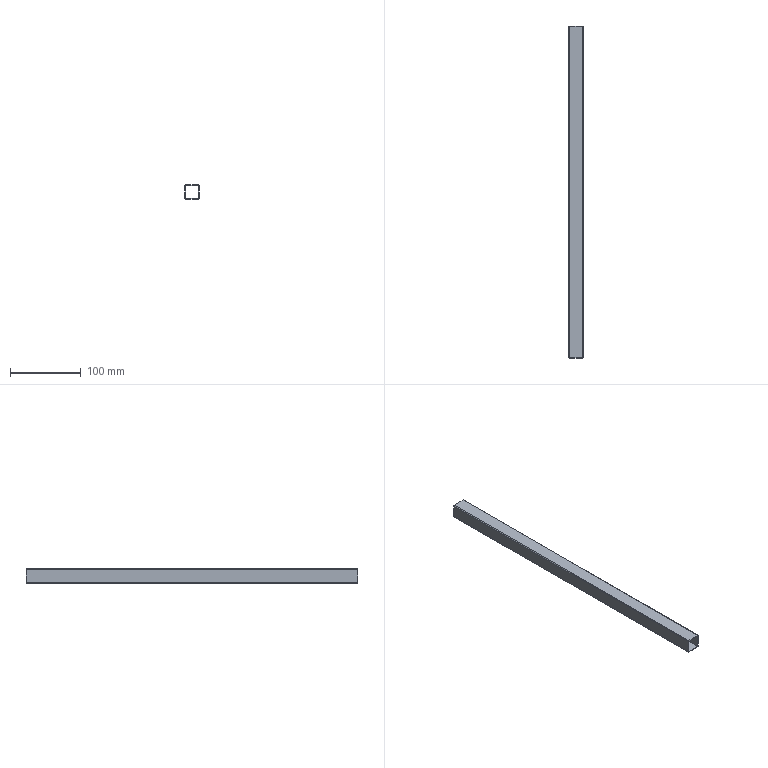Component | SolidWorks | DrawerStiffenerHorizontal-2 | 1 solid | 14 faces | box 20 x 470 x 20 mm | volume 42009 mm3 | plane 10 | cylinder 4 | commonest cylinder face diameters 2 x4
build123d program:
from build123d import *

# Parameters (mm, degrees)
SKETCH1_W           = 17.6
SKETCH1_H           = 17.6
BOSS_EXTRUDE1_DEPTH = 470


with BuildPart() as part:
    # Sketch1 → Boss-Extrude1 (new body)
    with BuildSketch(Plane.XY):
        with BuildLine():
            Line((-9, 10), (9, 10))
            ThreePointArc((9, 10), (9.707, 9.707), (10, 9))
            Line((10, 9), (10, -9))
            ThreePointArc((10, -9), (9.707, -9.707), (9, -10))
            Line((9, -10), (-9, -10))
            ThreePointArc((-9, -10), (-9.707, -9.707), (-10, -9))
            Line((-10, -9), (-10, 9))
            ThreePointArc((-10, 9), (-9.707, 9.707), (-9, 10))
        make_face()
        Rectangle(SKETCH1_W, SKETCH1_H, mode=Mode.SUBTRACT)
    extrude(amount=BOSS_EXTRUDE1_DEPTH)


solid = part.part

# Placed as in the assembly
solid = solid.moved(Location((8.5, 236, 110), (90, 0, 0)))
STEP:
#1=CARTESIAN_POINT('',(0.7283,-9.213,4.685));
#2=VERTEX_POINT('',#1);
#3=CARTESIAN_POINT('',(0.689,-9.213,4.724));
#4=VERTEX_POINT('',#3);
#5=CARTESIAN_POINT('',(0.689,-9.213,4.685));
#6=DIRECTION('',(-0.,-1.,-0.));
#7=DIRECTION('',(0.,0.,-1.));
#8=AXIS2_PLACEMENT_3D('',#5,#6,#7);
#9=CIRCLE('',#8,0.03937);
#10=EDGE_CURVE('',#2,#4,#9,.T.);
#11=ORIENTED_EDGE('',*,*,#10,.T.);
#12=CARTESIAN_POINT('',(-0.01969,-9.213,4.724));
#13=VERTEX_POINT('',#12);
#14=CARTESIAN_POINT('',(0.689,-9.213,4.724));
#15=DIRECTION('',(-1.,-0.,-0.));
#16=VECTOR('',#15,39.37);
#17=LINE('',#14,#16);
#18=EDGE_CURVE('',#4,#13,#17,.T.);
#19=ORIENTED_EDGE('',*,*,#18,.T.);
#20=CARTESIAN_POINT('',(-0.05906,-9.213,4.685));
#21=VERTEX_POINT('',#20);
#22=CARTESIAN_POINT('',(-0.01969,-9.213,4.685));
#23=DIRECTION('',(-0.,-1.,-0.));
#24=DIRECTION('',(0.,0.,1.));
#25=AXIS2_PLACEMENT_3D('',#22,#23,#24);
#26=CIRCLE('',#25,0.03937);
#27=EDGE_CURVE('',#13,#21,#26,.T.);
#28=ORIENTED_EDGE('',*,*,#27,.T.);
#29=CARTESIAN_POINT('',(-0.05906,-9.213,3.976));
#30=VERTEX_POINT('',#29);
#31=CARTESIAN_POINT('',(-0.05906,-9.213,4.685));
#32=DIRECTION('',(-0.,0.,-1.));
#33=VECTOR('',#32,39.37);
#34=LINE('',#31,#33);
#35=EDGE_CURVE('',#21,#30,#34,.T.);
#36=ORIENTED_EDGE('',*,*,#35,.T.);
#37=CARTESIAN_POINT('',(-0.01969,-9.213,3.937));
#38=VERTEX_POINT('',#37);
#39=CARTESIAN_POINT('',(-0.01969,-9.213,3.976));
#40=DIRECTION('',(-0.,-1.,-0.));
#41=DIRECTION('',(0.,0.,-1.));
#42=AXIS2_PLACEMENT_3D('',#39,#40,#41);
#43=CIRCLE('',#42,0.03937);
#44=EDGE_CURVE('',#30,#38,#43,.T.);
#45=ORIENTED_EDGE('',*,*,#44,.T.);
#46=CARTESIAN_POINT('',(0.689,-9.213,3.937));
#47=VERTEX_POINT('',#46);
#48=CARTESIAN_POINT('',(0.689,-9.213,3.937));
#49=DIRECTION('',(1.,0.,0.));
#50=VECTOR('',#49,39.37);
#51=LINE('',#48,#50);
#52=EDGE_CURVE('',#38,#47,#51,.T.);
#53=ORIENTED_EDGE('',*,*,#52,.T.);
#54=CARTESIAN_POINT('',(0.7283,-9.213,3.976));
#55=VERTEX_POINT('',#54);
#56=CARTESIAN_POINT('',(0.689,-9.213,3.976));
#57=DIRECTION('',(-0.,-1.,-0.));
#58=DIRECTION('',(0.,0.,-1.));
#59=AXIS2_PLACEMENT_3D('',#56,#57,#58);
#60=CIRCLE('',#59,0.03937);
#61=EDGE_CURVE('',#47,#55,#60,.T.);
#62=ORIENTED_EDGE('',*,*,#61,.T.);
#63=CARTESIAN_POINT('',(0.7283,-9.213,4.685));
#64=DIRECTION('',(0.,-0.,1.));
#65=VECTOR('',#64,39.37);
#66=LINE('',#63,#65);
#67=EDGE_CURVE('',#55,#2,#66,.T.);
#68=ORIENTED_EDGE('',*,*,#67,.T.);
#69=EDGE_LOOP('',(#11,#19,#28,#36,#45,#53,#62,#68));
#70=FACE_OUTER_BOUND('',#69,.T.);
#71=CARTESIAN_POINT('',(0.6811,-9.213,4.677));
#72=VERTEX_POINT('',#71);
#73=CARTESIAN_POINT('',(-0.01181,-9.213,4.677));
#74=VERTEX_POINT('',#73);
#75=CARTESIAN_POINT('',(0.6811,-9.213,4.677));
#76=DIRECTION('',(-1.,-0.,-0.));
#77=VECTOR('',#76,39.37);
#78=LINE('',#75,#77);
#79=EDGE_CURVE('',#72,#74,#78,.T.);
#80=ORIENTED_EDGE('',*,*,#79,.F.);
#81=CARTESIAN_POINT('',(0.6811,-9.213,3.984));
#82=VERTEX_POINT('',#81);
#83=CARTESIAN_POINT('',(0.6811,-9.213,4.677));
#84=DIRECTION('',(0.,-0.,1.));
#85=VECTOR('',#84,39.37);
#86=LINE('',#83,#85);
#87=EDGE_CURVE('',#82,#72,#86,.T.);
#88=ORIENTED_EDGE('',*,*,#87,.F.);
#89=CARTESIAN_POINT('',(-0.01181,-9.213,3.984));
#90=VERTEX_POINT('',#89);
#91=CARTESIAN_POINT('',(0.6811,-9.213,3.984));
#92=DIRECTION('',(1.,0.,0.));
#93=VECTOR('',#92,39.37);
#94=LINE('',#91,#93);
#95=EDGE_CURVE('',#90,#82,#94,.T.);
#96=ORIENTED_EDGE('',*,*,#95,.F.);
#97=CARTESIAN_POINT('',(-0.01181,-9.213,4.677));
#98=DIRECTION('',(-0.,0.,-1.));
#99=VECTOR('',#98,39.37);
#100=LINE('',#97,#99);
#101=EDGE_CURVE('',#74,#90,#100,.T.);
#102=ORIENTED_EDGE('',*,*,#101,.F.);
#103=EDGE_LOOP('',(#80,#88,#96,#102));
#104=FACE_BOUND('',#103,.T.);
#105=CARTESIAN_POINT('',(0.689,-9.213,4.685));
#106=DIRECTION('',(-0.,-1.,-0.));
#107=DIRECTION('',(-0.,0.,-1.));
#108=AXIS2_PLACEMENT_3D('',#105,#106,#107);
#109=PLANE('',#108);
#110=ADVANCED_FACE('',(#70,#104),#109,.T.);
#111=CARTESIAN_POINT('',(0.7283,9.291,4.685));
#112=VERTEX_POINT('',#111);
#113=CARTESIAN_POINT('',(0.689,9.291,4.724));
#114=VERTEX_POINT('',#113);
#115=CARTESIAN_POINT('',(0.689,9.291,4.685));
#116=DIRECTION('',(-0.,-1.,-0.));
#117=DIRECTION('',(0.,0.,-1.));
#118=AXIS2_PLACEMENT_3D('',#115,#116,#117);
#119=CIRCLE('',#118,0.03937);
#120=EDGE_CURVE('',#112,#114,#119,.T.);
#121=ORIENTED_EDGE('',*,*,#120,.F.);
#122=CARTESIAN_POINT('',(0.7283,9.291,3.976));
#123=VERTEX_POINT('',#122);
#124=CARTESIAN_POINT('',(0.7283,9.291,4.685));
#125=DIRECTION('',(0.,-0.,1.));
#126=VECTOR('',#125,39.37);
#127=LINE('',#124,#126);
#128=EDGE_CURVE('',#123,#112,#127,.T.);
#129=ORIENTED_EDGE('',*,*,#128,.F.);
#130=CARTESIAN_POINT('',(0.689,9.291,3.937));
#131=VERTEX_POINT('',#130);
#132=CARTESIAN_POINT('',(0.689,9.291,3.976));
#133=DIRECTION('',(-0.,-1.,-0.));
#134=DIRECTION('',(0.,0.,-1.));
#135=AXIS2_PLACEMENT_3D('',#132,#133,#134);
#136=CIRCLE('',#135,0.03937);
#137=EDGE_CURVE('',#131,#123,#136,.T.);
#138=ORIENTED_EDGE('',*,*,#137,.F.);
#139=CARTESIAN_POINT('',(-0.01969,9.291,3.937));
#140=VERTEX_POINT('',#139);
#141=CARTESIAN_POINT('',(0.689,9.291,3.937));
#142=DIRECTION('',(1.,0.,0.));
#143=VECTOR('',#142,39.37);
#144=LINE('',#141,#143);
#145=EDGE_CURVE('',#140,#131,#144,.T.);
#146=ORIENTED_EDGE('',*,*,#145,.F.);
#147=CARTESIAN_POINT('',(-0.05906,9.291,3.976));
#148=VERTEX_POINT('',#147);
#149=CARTESIAN_POINT('',(-0.01969,9.291,3.976));
#150=DIRECTION('',(-0.,-1.,-0.));
#151=DIRECTION('',(0.,0.,-1.));
#152=AXIS2_PLACEMENT_3D('',#149,#150,#151);
#153=CIRCLE('',#152,0.03937);
#154=EDGE_CURVE('',#148,#140,#153,.T.);
#155=ORIENTED_EDGE('',*,*,#154,.F.);
#156=CARTESIAN_POINT('',(-0.05906,9.291,4.685));
#157=VERTEX_POINT('',#156);
#158=CARTESIAN_POINT('',(-0.05906,9.291,4.685));
#159=DIRECTION('',(-0.,0.,-1.));
#160=VECTOR('',#159,39.37);
#161=LINE('',#158,#160);
#162=EDGE_CURVE('',#157,#148,#161,.T.);
#163=ORIENTED_EDGE('',*,*,#162,.F.);
#164=CARTESIAN_POINT('',(-0.01969,9.291,4.724));
#165=VERTEX_POINT('',#164);
#166=CARTESIAN_POINT('',(-0.01969,9.291,4.685));
#167=DIRECTION('',(-0.,-1.,-0.));
#168=DIRECTION('',(0.,0.,1.));
#169=AXIS2_PLACEMENT_3D('',#166,#167,#168);
#170=CIRCLE('',#169,0.03937);
#171=EDGE_CURVE('',#165,#157,#170,.T.);
#172=ORIENTED_EDGE('',*,*,#171,.F.);
#173=CARTESIAN_POINT('',(0.689,9.291,4.724));
#174=DIRECTION('',(-1.,-0.,-0.));
#175=VECTOR('',#174,39.37);
#176=LINE('',#173,#175);
#177=EDGE_CURVE('',#114,#165,#176,.T.);
#178=ORIENTED_EDGE('',*,*,#177,.F.);
#179=EDGE_LOOP('',(#121,#129,#138,#146,#155,#163,#172,#178));
#180=FACE_OUTER_BOUND('',#179,.T.);
#181=CARTESIAN_POINT('',(0.6811,9.291,3.984));
#182=VERTEX_POINT('',#181);
#183=CARTESIAN_POINT('',(0.6811,9.291,4.677));
#184=VERTEX_POINT('',#183);
#185=CARTESIAN_POINT('',(0.6811,9.291,4.677));
#186=DIRECTION('',(0.,-0.,1.));
#187=VECTOR('',#186,39.37);
#188=LINE('',#185,#187);
#189=EDGE_CURVE('',#182,#184,#188,.T.);
#190=ORIENTED_EDGE('',*,*,#189,.T.);
#191=CARTESIAN_POINT('',(-0.01181,9.291,4.677));
#192=VERTEX_POINT('',#191);
#193=CARTESIAN_POINT('',(0.6811,9.291,4.677));
#194=DIRECTION('',(-1.,-0.,-0.));
#195=VECTOR('',#194,39.37);
#196=LINE('',#193,#195);
#197=EDGE_CURVE('',#184,#192,#196,.T.);
#198=ORIENTED_EDGE('',*,*,#197,.T.);
#199=CARTESIAN_POINT('',(-0.01181,9.291,3.984));
#200=VERTEX_POINT('',#199);
#201=CARTESIAN_POINT('',(-0.01181,9.291,4.677));
#202=DIRECTION('',(-0.,0.,-1.));
#203=VECTOR('',#202,39.37);
#204=LINE('',#201,#203);
#205=EDGE_CURVE('',#192,#200,#204,.T.);
#206=ORIENTED_EDGE('',*,*,#205,.T.);
#207=CARTESIAN_POINT('',(0.6811,9.291,3.984));
#208=DIRECTION('',(1.,0.,0.));
#209=VECTOR('',#208,39.37);
#210=LINE('',#207,#209);
#211=EDGE_CURVE('',#200,#182,#210,.T.);
#212=ORIENTED_EDGE('',*,*,#211,.T.);
#213=EDGE_LOOP('',(#190,#198,#206,#212));
#214=FACE_BOUND('',#213,.T.);
#215=CARTESIAN_POINT('',(0.689,9.291,4.685));
#216=DIRECTION('',(-0.,-1.,-0.));
#217=DIRECTION('',(-0.,0.,-1.));
#218=AXIS2_PLACEMENT_3D('',#215,#216,#217);
#219=PLANE('',#218);
#220=ADVANCED_FACE('',(#180,#214),#219,.F.);
#221=ORIENTED_EDGE('',*,*,#120,.T.);
#222=CARTESIAN_POINT('',(0.689,-9.213,4.724));
#223=DIRECTION('',(0.,1.,0.));
#224=VECTOR('',#223,39.37);
#225=LINE('',#222,#224);
#226=EDGE_CURVE('',#4,#114,#225,.T.);
#227=ORIENTED_EDGE('',*,*,#226,.F.);
#228=ORIENTED_EDGE('',*,*,#10,.F.);
#229=CARTESIAN_POINT('',(0.7283,-9.213,4.685));
#230=DIRECTION('',(0.,1.,0.));
#231=VECTOR('',#230,39.37);
#232=LINE('',#229,#231);
#233=EDGE_CURVE('',#2,#112,#232,.T.);
#234=ORIENTED_EDGE('',*,*,#233,.T.);
#235=EDGE_LOOP('',(#221,#227,#228,#234));
#236=FACE_OUTER_BOUND('',#235,.T.);
#237=CARTESIAN_POINT('',(0.689,-9.213,4.685));
#238=DIRECTION('',(0.,1.,0.));
#239=DIRECTION('',(0.,0.,1.));
#240=AXIS2_PLACEMENT_3D('',#237,#238,#239);
#241=CYLINDRICAL_SURFACE('',#240,0.03937);
#242=ADVANCED_FACE('',(#236),#241,.T.);
#243=ORIENTED_EDGE('',*,*,#177,.T.);
#244=CARTESIAN_POINT('',(-0.01969,-9.213,4.724));
#245=DIRECTION('',(0.,1.,0.));
#246=VECTOR('',#245,39.37);
#247=LINE('',#244,#246);
#248=EDGE_CURVE('',#13,#165,#247,.T.);
#249=ORIENTED_EDGE('',*,*,#248,.F.);
#250=ORIENTED_EDGE('',*,*,#18,.F.);
#251=ORIENTED_EDGE('',*,*,#226,.T.);
#252=EDGE_LOOP('',(#243,#249,#250,#251));
#253=FACE_OUTER_BOUND('',#252,.T.);
#254=CARTESIAN_POINT('',(0.689,-9.213,4.724));
#255=DIRECTION('',(-0.,0.,-1.));
#256=DIRECTION('',(0.,1.,0.));
#257=AXIS2_PLACEMENT_3D('',#254,#255,#256);
#258=PLANE('',#257);
#259=ADVANCED_FACE('',(#253),#258,.F.);
#260=ORIENTED_EDGE('',*,*,#171,.T.);
#261=CARTESIAN_POINT('',(-0.05906,-9.213,4.685));
#262=DIRECTION('',(0.,1.,0.));
#263=VECTOR('',#262,39.37);
#264=LINE('',#261,#263);
#265=EDGE_CURVE('',#21,#157,#264,.T.);
#266=ORIENTED_EDGE('',*,*,#265,.F.);
#267=ORIENTED_EDGE('',*,*,#27,.F.);
#268=ORIENTED_EDGE('',*,*,#248,.T.);
#269=EDGE_LOOP('',(#260,#266,#267,#268));
#270=FACE_OUTER_BOUND('',#269,.T.);
#271=CARTESIAN_POINT('',(-0.01969,-9.213,4.685));
#272=DIRECTION('',(0.,1.,0.));
#273=DIRECTION('',(0.,0.,1.));
#274=AXIS2_PLACEMENT_3D('',#271,#272,#273);
#275=CYLINDRICAL_SURFACE('',#274,0.03937);
#276=ADVANCED_FACE('',(#270),#275,.T.);
#277=ORIENTED_EDGE('',*,*,#162,.T.);
#278=CARTESIAN_POINT('',(-0.05906,-9.213,3.976));
#279=DIRECTION('',(0.,1.,0.));
#280=VECTOR('',#279,39.37);
#281=LINE('',#278,#280);
#282=EDGE_CURVE('',#30,#148,#281,.T.);
#283=ORIENTED_EDGE('',*,*,#282,.F.);
#284=ORIENTED_EDGE('',*,*,#35,.F.);
#285=ORIENTED_EDGE('',*,*,#265,.T.);
#286=EDGE_LOOP('',(#277,#283,#284,#285));
#287=FACE_OUTER_BOUND('',#286,.T.);
#288=CARTESIAN_POINT('',(-0.05906,-9.213,4.685));
#289=DIRECTION('',(1.,-0.,0.));
#290=DIRECTION('',(-0.,-1.,-0.));
#291=AXIS2_PLACEMENT_3D('',#288,#289,#290);
#292=PLANE('',#291);
#293=ADVANCED_FACE('',(#287),#292,.F.);
#294=ORIENTED_EDGE('',*,*,#154,.T.);
#295=CARTESIAN_POINT('',(-0.01969,-9.213,3.937));
#296=DIRECTION('',(0.,1.,0.));
#297=VECTOR('',#296,39.37);
#298=LINE('',#295,#297);
#299=EDGE_CURVE('',#38,#140,#298,.T.);
#300=ORIENTED_EDGE('',*,*,#299,.F.);
#301=ORIENTED_EDGE('',*,*,#44,.F.);
#302=ORIENTED_EDGE('',*,*,#282,.T.);
#303=EDGE_LOOP('',(#294,#300,#301,#302));
#304=FACE_OUTER_BOUND('',#303,.T.);
#305=CARTESIAN_POINT('',(-0.01969,-9.213,3.976));
#306=DIRECTION('',(0.,1.,0.));
#307=DIRECTION('',(0.,0.,1.));
#308=AXIS2_PLACEMENT_3D('',#305,#306,#307);
#309=CYLINDRICAL_SURFACE('',#308,0.03937);
#310=ADVANCED_FACE('',(#304),#309,.T.);
#311=ORIENTED_EDGE('',*,*,#145,.T.);
#312=CARTESIAN_POINT('',(0.689,-9.213,3.937));
#313=DIRECTION('',(0.,1.,0.));
#314=VECTOR('',#313,39.37);
#315=LINE('',#312,#314);
#316=EDGE_CURVE('',#47,#131,#315,.T.);
#317=ORIENTED_EDGE('',*,*,#316,.F.);
#318=ORIENTED_EDGE('',*,*,#52,.F.);
#319=ORIENTED_EDGE('',*,*,#299,.T.);
#320=EDGE_LOOP('',(#311,#317,#318,#319));
#321=FACE_OUTER_BOUND('',#320,.T.);
#322=CARTESIAN_POINT('',(0.689,-9.213,3.937));
#323=DIRECTION('',(-0.,-0.,1.));
#324=DIRECTION('',(-1.,-0.,-0.));
#325=AXIS2_PLACEMENT_3D('',#322,#323,#324);
#326=PLANE('',#325);
#327=ADVANCED_FACE('',(#321),#326,.F.);
#328=ORIENTED_EDGE('',*,*,#137,.T.);
#329=CARTESIAN_POINT('',(0.7283,-9.213,3.976));
#330=DIRECTION('',(0.,1.,0.));
#331=VECTOR('',#330,39.37);
#332=LINE('',#329,#331);
#333=EDGE_CURVE('',#55,#123,#332,.T.);
#334=ORIENTED_EDGE('',*,*,#333,.F.);
#335=ORIENTED_EDGE('',*,*,#61,.F.);
#336=ORIENTED_EDGE('',*,*,#316,.T.);
#337=EDGE_LOOP('',(#328,#334,#335,#336));
#338=FACE_OUTER_BOUND('',#337,.T.);
#339=CARTESIAN_POINT('',(0.689,-9.213,3.976));
#340=DIRECTION('',(0.,1.,0.));
#341=DIRECTION('',(0.,0.,1.));
#342=AXIS2_PLACEMENT_3D('',#339,#340,#341);
#343=CYLINDRICAL_SURFACE('',#342,0.03937);
#344=ADVANCED_FACE('',(#338),#343,.T.);
#345=ORIENTED_EDGE('',*,*,#128,.T.);
#346=ORIENTED_EDGE('',*,*,#233,.F.);
#347=ORIENTED_EDGE('',*,*,#67,.F.);
#348=ORIENTED_EDGE('',*,*,#333,.T.);
#349=EDGE_LOOP('',(#345,#346,#347,#348));
#350=FACE_OUTER_BOUND('',#349,.T.);
#351=CARTESIAN_POINT('',(0.7283,-9.213,4.685));
#352=DIRECTION('',(-1.,0.,-0.));
#353=DIRECTION('',(0.,1.,0.));
#354=AXIS2_PLACEMENT_3D('',#351,#352,#353);
#355=PLANE('',#354);
#356=ADVANCED_FACE('',(#350),#355,.F.);
#357=ORIENTED_EDGE('',*,*,#189,.F.);
#358=CARTESIAN_POINT('',(0.6811,-9.213,3.984));
#359=DIRECTION('',(0.,1.,0.));
#360=VECTOR('',#359,39.37);
#361=LINE('',#358,#360);
#362=EDGE_CURVE('',#82,#182,#361,.T.);
#363=ORIENTED_EDGE('',*,*,#362,.F.);
#364=ORIENTED_EDGE('',*,*,#87,.T.);
#365=CARTESIAN_POINT('',(0.6811,-9.213,4.677));
#366=DIRECTION('',(0.,1.,0.));
#367=VECTOR('',#366,39.37);
#368=LINE('',#365,#367);
#369=EDGE_CURVE('',#72,#184,#368,.T.);
#370=ORIENTED_EDGE('',*,*,#369,.T.);
#371=EDGE_LOOP('',(#357,#363,#364,#370));
#372=FACE_OUTER_BOUND('',#371,.T.);
#373=CARTESIAN_POINT('',(0.6811,-9.213,4.677));
#374=DIRECTION('',(-1.,0.,-0.));
#375=DIRECTION('',(0.,1.,0.));
#376=AXIS2_PLACEMENT_3D('',#373,#374,#375);
#377=PLANE('',#376);
#378=ADVANCED_FACE('',(#372),#377,.T.);
#379=ORIENTED_EDGE('',*,*,#197,.F.);
#380=ORIENTED_EDGE('',*,*,#369,.F.);
#381=ORIENTED_EDGE('',*,*,#79,.T.);
#382=CARTESIAN_POINT('',(-0.01181,-9.213,4.677));
#383=DIRECTION('',(0.,1.,0.));
#384=VECTOR('',#383,39.37);
#385=LINE('',#382,#384);
#386=EDGE_CURVE('',#74,#192,#385,.T.);
#387=ORIENTED_EDGE('',*,*,#386,.T.);
#388=EDGE_LOOP('',(#379,#380,#381,#387));
#389=FACE_OUTER_BOUND('',#388,.T.);
#390=CARTESIAN_POINT('',(0.6811,-9.213,4.677));
#391=DIRECTION('',(0.,0.,-1.));
#392=DIRECTION('',(1.,0.,0.));
#393=AXIS2_PLACEMENT_3D('',#390,#391,#392);
#394=PLANE('',#393);
#395=ADVANCED_FACE('',(#389),#394,.T.);
#396=ORIENTED_EDGE('',*,*,#205,.F.);
#397=ORIENTED_EDGE('',*,*,#386,.F.);
#398=ORIENTED_EDGE('',*,*,#101,.T.);
#399=CARTESIAN_POINT('',(-0.01181,-9.213,3.984));
#400=DIRECTION('',(0.,1.,0.));
#401=VECTOR('',#400,39.37);
#402=LINE('',#399,#401);
#403=EDGE_CURVE('',#90,#200,#402,.T.);
#404=ORIENTED_EDGE('',*,*,#403,.T.);
#405=EDGE_LOOP('',(#396,#397,#398,#404));
#406=FACE_OUTER_BOUND('',#405,.T.);
#407=CARTESIAN_POINT('',(-0.01181,-9.213,4.677));
#408=DIRECTION('',(1.,-0.,0.));
#409=DIRECTION('',(-0.,-1.,-0.));
#410=AXIS2_PLACEMENT_3D('',#407,#408,#409);
#411=PLANE('',#410);
#412=ADVANCED_FACE('',(#406),#411,.T.);
#413=ORIENTED_EDGE('',*,*,#211,.F.);
#414=ORIENTED_EDGE('',*,*,#403,.F.);
#415=ORIENTED_EDGE('',*,*,#95,.T.);
#416=ORIENTED_EDGE('',*,*,#362,.T.);
#417=EDGE_LOOP('',(#413,#414,#415,#416));
#418=FACE_OUTER_BOUND('',#417,.T.);
#419=CARTESIAN_POINT('',(0.6811,-9.213,3.984));
#420=DIRECTION('',(-0.,-0.,1.));
#421=DIRECTION('',(-1.,-0.,-0.));
#422=AXIS2_PLACEMENT_3D('',#419,#420,#421);
#423=PLANE('',#422);
#424=ADVANCED_FACE('',(#418),#423,.T.);
#425=CLOSED_SHELL('',(#110,#220,#242,#259,#276,#293,#310,#327,#344,#356,#378,#395,#412,#424));
#426=MANIFOLD_SOLID_BREP('',#425);
#427=CARTESIAN_POINT('',(0.,0.,0.));
#428=DIRECTION('',(0.,0.,1.));
#429=DIRECTION('',(1.,0.,0.));
#430=AXIS2_PLACEMENT_3D('',#427,#428,#429);
#431=(LENGTH_UNIT()NAMED_UNIT(*)SI_UNIT($,.METRE.));
#432=LENGTH_MEASURE_WITH_UNIT(LENGTH_MEASURE(0.0254),#431);
#433=DIMENSIONAL_EXPONENTS(1.,0.,0.,0.,0.,0.,0.);
#434=(CONVERSION_BASED_UNIT('',#432)LENGTH_UNIT()NAMED_UNIT(#433));
#435=UNCERTAINTY_MEASURE_WITH_UNIT(LENGTH_MEASURE(0.00001),#434,'','');
#436=(NAMED_UNIT(*)PLANE_ANGLE_UNIT()SI_UNIT($,.RADIAN.));
#437=(NAMED_UNIT(*)SI_UNIT($,.STERADIAN.)SOLID_ANGLE_UNIT());
#438=(GEOMETRIC_REPRESENTATION_CONTEXT(3)GLOBAL_UNCERTAINTY_ASSIGNED_CONTEXT((#435))GLOBAL_UNIT_ASSIGNED_CONTEXT((#434,#436,#437))REPRESENTATION_CONTEXT('',''));
#439=ADVANCED_BREP_SHAPE_REPRESENTATION('',(#426,#430),#438);
#440=COLOUR_RGB('',0.7922,0.8196,0.9333);
#441=FILL_AREA_STYLE_COLOUR('',#440);
#442=FILL_AREA_STYLE('',(#441));
#443=SURFACE_STYLE_FILL_AREA(#442);
#444=SURFACE_SIDE_STYLE('',(#443));
#445=SURFACE_STYLE_USAGE(.BOTH.,#444);
#446=PRESENTATION_STYLE_ASSIGNMENT((#445));
#447=STYLED_ITEM('',(#446),#426);
#448=PRESENTATION_LAYER_ASSIGNMENT('','',(#447));
#449=(LENGTH_UNIT()NAMED_UNIT(*)SI_UNIT($,.METRE.));
#450=LENGTH_MEASURE_WITH_UNIT(LENGTH_MEASURE(0.0254),#449);
#451=DIMENSIONAL_EXPONENTS(1.,0.,0.,0.,0.,0.,0.);
#452=(CONVERSION_BASED_UNIT('',#450)LENGTH_UNIT()NAMED_UNIT(#451));
#453=UNCERTAINTY_MEASURE_WITH_UNIT(LENGTH_MEASURE(0.00001),#452,'','');
#454=(NAMED_UNIT(*)PLANE_ANGLE_UNIT()SI_UNIT($,.RADIAN.));
#455=(NAMED_UNIT(*)SI_UNIT($,.STERADIAN.)SOLID_ANGLE_UNIT());
#456=(GEOMETRIC_REPRESENTATION_CONTEXT(3)GLOBAL_UNCERTAINTY_ASSIGNED_CONTEXT((#453))GLOBAL_UNIT_ASSIGNED_CONTEXT((#452,#454,#455))REPRESENTATION_CONTEXT('',''));
#457=MECHANICAL_DESIGN_GEOMETRIC_PRESENTATION_REPRESENTATION('',(#447),#456);